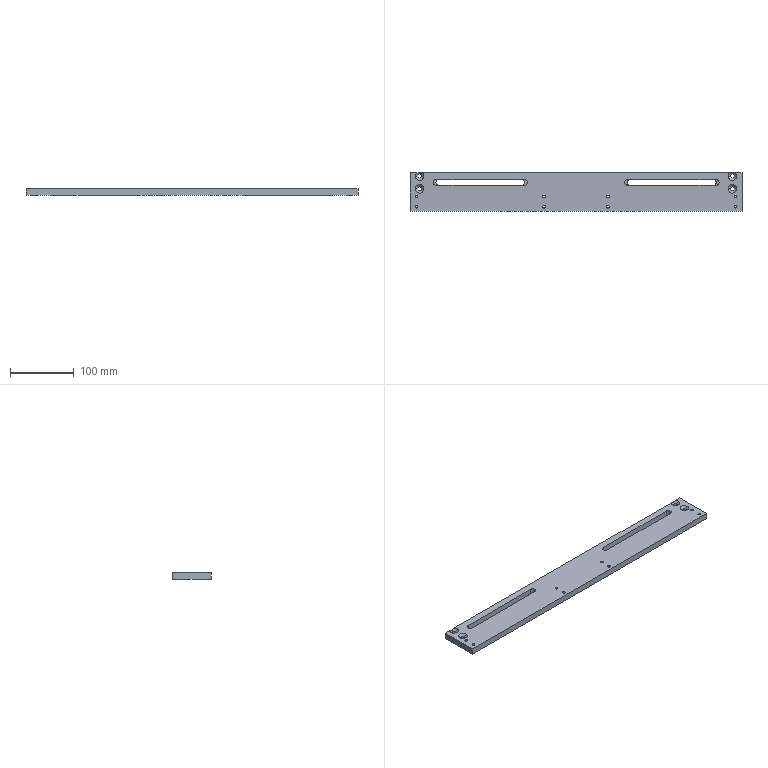Component | SolidWorks | GuideWheelAdjustingPlate1-1 | 1 solid | 58 faces | box 520 x 60 x 10 mm | volume 282862 mm3 | cylinder 36 | plane 14 | cone 8 | commonest cylinder face diameters 4.2 x16 9 x12 6.5 x8
build123d program:
from build123d import *

# Parameters (mm, degrees)
SKETCH1_2_W                                          = 520
SKETCH1_2_H                                          = 30
BOSS_EXTRUDE1_DEPTH                                  = 10
CUT_EXTRUDE1_DEPTH                                   = 261.624
SKETCH3_W                                            = 520
SKETCH3_H                                            = 10
BOSS_EXTRUDE2_DEPTH                                  = 30
M5_TAPPED_HOLE1_D                                    = 4.2
COUNTERSUNK_HOLE_1_FOR_M6_HEX_SOCKET_COU_D           = 6.5
COUNTERSUNK_HOLE_1_FOR_M6_HEX_SOCKET_COU_CSINK_D     = 13.44
COUNTERSUNK_HOLE_1_FOR_M6_HEX_SOCKET_COU_CSINK_ANGLE = 90
SLOTENDRELIEF_DEPTH                                  = 8.5


with BuildPart() as part:
    # Sketch1_2 → Boss-Extrude1 (new body)
    with BuildSketch(Plane.XY):
        Rectangle(SKETCH1_2_W, SKETCH1_2_H)
    extrude(amount=BOSS_EXTRUDE1_DEPTH)

    # Sketch2 → Cut-Extrude1 (cut, through all)
    with BuildSketch(Plane.XY.offset(10)):
        with BuildLine():
            Line((-215, 4.5), (-85, 4.5))
            ThreePointArc((-85, 4.5), (-80.5, 0), (-85, -4.5))
            Line((-85, -4.5), (-215, -4.5))
            ThreePointArc((-215, -4.5), (-219.5, 0), (-215, 4.5))
        make_face()
        with BuildLine():
            Line((215, 4.5), (85, 4.5))
            ThreePointArc((85, 4.5), (80.5, 0), (85, -4.5))
            Line((85, -4.5), (215, -4.5))
            ThreePointArc((215, -4.5), (219.5, 0), (215, 4.5))
        make_face()
    extrude(amount=-CUT_EXTRUDE1_DEPTH, mode=Mode.SUBTRACT)

    # Sketch3 → Boss-Extrude2 (add)
    with BuildSketch(Plane.XZ.offset(15)):
        with Locations((0, 5)):
            Rectangle(SKETCH3_W, SKETCH3_H)
    extrude(amount=BOSS_EXTRUDE2_DEPTH)

    # M5 Tapped Hole1 (through all)
    with Locations(Plane.XY.offset(10)):
        with Locations((-250, -22), (-250, -38), (-50, -22), (-50, -38), (50, -22), (50, -38), (250, -22), (250, -38)):
            Hole(M5_TAPPED_HOLE1_D / 2)

    # Countersunk Hole 1 for M6 Hex Socket Cou (through all)
    with Locations(Plane.XY.offset(10)):
        with Locations((-245, -10), (-245, 10), (245, 10), (245, -10)):
            CounterSinkHole(COUNTERSUNK_HOLE_1_FOR_M6_HEX_SOCKET_COU_D / 2, COUNTERSUNK_HOLE_1_FOR_M6_HEX_SOCKET_COU_CSINK_D / 2, counter_sink_angle=COUNTERSUNK_HOLE_1_FOR_M6_HEX_SOCKET_COU_CSINK_ANGLE)

    # Sketch1 → SlotEndRelief (cut)
    with BuildSketch(Plane.XY.offset(10)):
        with BuildLine():
            Line((-215, 4.5), (-219.5, 4.5))
            ThreePointArc((-219.5, 4.5), (-224, 0), (-219.5, -4.5))
            Line((-219.5, -4.5), (-215, -4.5))
            Line((-215, -4.5), (-215, 4.5))
        make_face()
        with BuildLine():
            Line((-85, 4.5), (-80.5, 4.5))
            ThreePointArc((-80.5, 4.5), (-76, 0), (-80.5, -4.5))
            Line((-80.5, -4.5), (-85, -4.5))
            Line((-85, -4.5), (-85, 4.5))
        make_face()
        with BuildLine():
            Line((85, 4.5), (80.5, 4.5))
            ThreePointArc((80.5, 4.5), (76, 0), (80.5, -4.5))
            Line((80.5, -4.5), (85, -4.5))
            Line((85, -4.5), (85, 4.5))
        make_face()
        with BuildLine():
            Line((215, 4.5), (219.5, 4.5))
            ThreePointArc((219.5, 4.5), (224, 0), (219.5, -4.5))
            Line((219.5, -4.5), (215, -4.5))
            Line((215, -4.5), (215, 4.5))
        make_face()
    extrude(amount=-SLOTENDRELIEF_DEPTH, mode=Mode.SUBTRACT)


solid = part.part

# Placed as in the assembly
solid = solid.moved(Location((-394.97, -65, 0), (0, 0, 0)))